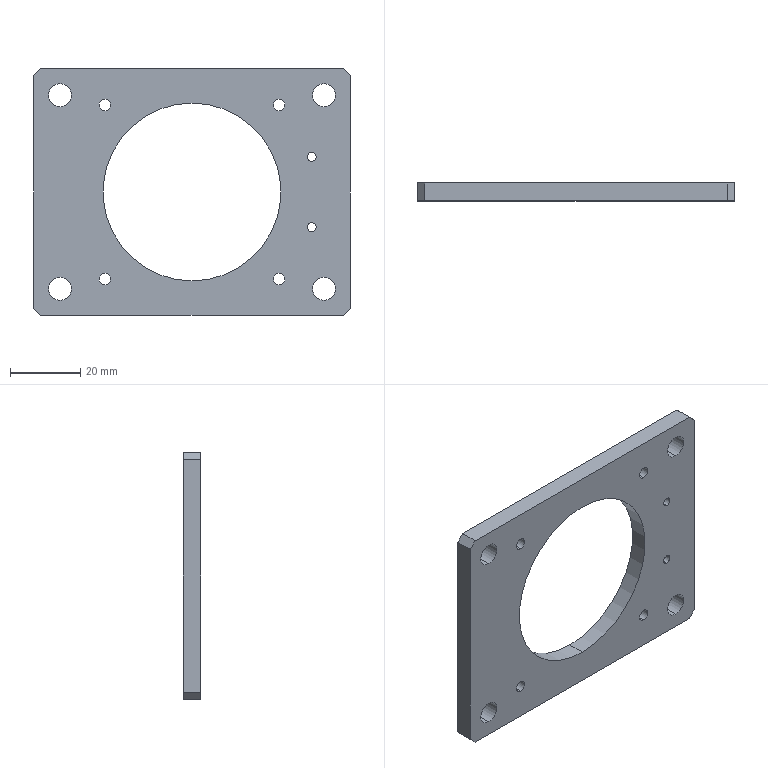Component | SolidWorks | H2020022-0411-1-1 | 1 solid | 32 faces | box 90 x 5 x 70 mm | volume 20561 mm3 | cylinder 22 | plane 10 | commonest cylinder face diameters 3.3 x8 6.5 x8 2.5 x4 50.5 x2 | material Stainless Steel304
STEP:
#1=COLOUR_RGB('',0.7922,0.8196,0.9333);
#2=FILL_AREA_STYLE_COLOUR('',#1);
#3=FILL_AREA_STYLE('',(#2));
#4=SURFACE_STYLE_FILL_AREA(#3);
#5=SURFACE_SIDE_STYLE('',(#4));
#6=SURFACE_STYLE_USAGE(.BOTH.,#5);
#7=PRESENTATION_STYLE_ASSIGNMENT((#6));
#8=CARTESIAN_POINT('',(0.1195,1.654,11.376));
#9=VERTEX_POINT('',#8);
#10=CARTESIAN_POINT('',(0.1195,1.654,11.474));
#11=VERTEX_POINT('',#10);
#12=CARTESIAN_POINT('',(0.1195,1.654,11.425));
#13=DIRECTION('',(0.,1.,-0.));
#14=DIRECTION('',(0.,0.,1.));
#15=AXIS2_PLACEMENT_3D('',#12,#13,#14);
#16=CIRCLE('',#15,0.04921);
#17=EDGE_CURVE('',#9,#11,#16,.T.);
#18=ORIENTED_EDGE('',*,*,#17,.F.);
#19=CARTESIAN_POINT('',(0.1195,1.851,11.376));
#20=VERTEX_POINT('',#19);
#21=CARTESIAN_POINT('',(0.1195,1.851,11.376));
#22=DIRECTION('',(0.,1.,-0.));
#23=VECTOR('',#22,39.37);
#24=LINE('',#21,#23);
#25=EDGE_CURVE('',#9,#20,#24,.T.);
#26=ORIENTED_EDGE('',*,*,#25,.T.);
#27=CARTESIAN_POINT('',(0.1195,1.851,11.474));
#28=VERTEX_POINT('',#27);
#29=CARTESIAN_POINT('',(0.1195,1.851,11.425));
#30=DIRECTION('',(0.,1.,-0.));
#31=DIRECTION('',(0.,0.,1.));
#32=AXIS2_PLACEMENT_3D('',#29,#30,#31);
#33=CIRCLE('',#32,0.04921);
#34=EDGE_CURVE('',#20,#28,#33,.T.);
#35=ORIENTED_EDGE('',*,*,#34,.T.);
#36=CARTESIAN_POINT('',(0.1195,1.851,11.474));
#37=DIRECTION('',(0.,1.,-0.));
#38=VECTOR('',#37,39.37);
#39=LINE('',#36,#38);
#40=EDGE_CURVE('',#11,#28,#39,.T.);
#41=ORIENTED_EDGE('',*,*,#40,.F.);
#42=EDGE_LOOP('',(#18,#26,#35,#41));
#43=FACE_OUTER_BOUND('',#42,.T.);
#44=CARTESIAN_POINT('',(0.1195,1.851,11.425));
#45=DIRECTION('',(0.,1.,-0.));
#46=DIRECTION('',(0.,0.,1.));
#47=AXIS2_PLACEMENT_3D('',#44,#45,#46);
#48=CYLINDRICAL_SURFACE('',#47,0.04921);
#49=ADVANCED_FACE('',(#43),#48,.F.);
#50=CARTESIAN_POINT('',(0.1195,1.654,10.588));
#51=VERTEX_POINT('',#50);
#52=CARTESIAN_POINT('',(0.1195,1.654,10.687));
#53=VERTEX_POINT('',#52);
#54=CARTESIAN_POINT('',(0.1195,1.654,10.638));
#55=DIRECTION('',(0.,1.,-0.));
#56=DIRECTION('',(0.,0.,1.));
#57=AXIS2_PLACEMENT_3D('',#54,#55,#56);
#58=CIRCLE('',#57,0.04921);
#59=EDGE_CURVE('',#51,#53,#58,.T.);
#60=ORIENTED_EDGE('',*,*,#59,.F.);
#61=CARTESIAN_POINT('',(0.1195,1.851,10.588));
#62=VERTEX_POINT('',#61);
#63=CARTESIAN_POINT('',(0.1195,1.851,10.588));
#64=DIRECTION('',(0.,1.,-0.));
#65=VECTOR('',#64,39.37);
#66=LINE('',#63,#65);
#67=EDGE_CURVE('',#51,#62,#66,.T.);
#68=ORIENTED_EDGE('',*,*,#67,.T.);
#69=CARTESIAN_POINT('',(0.1195,1.851,10.687));
#70=VERTEX_POINT('',#69);
#71=CARTESIAN_POINT('',(0.1195,1.851,10.638));
#72=DIRECTION('',(0.,1.,-0.));
#73=DIRECTION('',(0.,0.,1.));
#74=AXIS2_PLACEMENT_3D('',#71,#72,#73);
#75=CIRCLE('',#74,0.04921);
#76=EDGE_CURVE('',#62,#70,#75,.T.);
#77=ORIENTED_EDGE('',*,*,#76,.T.);
#78=CARTESIAN_POINT('',(0.1195,1.851,10.687));
#79=DIRECTION('',(0.,1.,-0.));
#80=VECTOR('',#79,39.37);
#81=LINE('',#78,#80);
#82=EDGE_CURVE('',#53,#70,#81,.T.);
#83=ORIENTED_EDGE('',*,*,#82,.F.);
#84=EDGE_LOOP('',(#60,#68,#77,#83));
#85=FACE_OUTER_BOUND('',#84,.T.);
#86=CARTESIAN_POINT('',(0.1195,1.851,10.638));
#87=DIRECTION('',(0.,1.,-0.));
#88=DIRECTION('',(0.,0.,1.));
#89=AXIS2_PLACEMENT_3D('',#86,#87,#88);
#90=CYLINDRICAL_SURFACE('',#89,0.04921);
#91=ADVANCED_FACE('',(#85),#90,.F.);
#92=CARTESIAN_POINT('',(-2.193,1.654,12.071));
#93=VERTEX_POINT('',#92);
#94=CARTESIAN_POINT('',(-2.193,1.654,11.941));
#95=VERTEX_POINT('',#94);
#96=CARTESIAN_POINT('',(-2.193,1.654,12.006));
#97=DIRECTION('',(-0.,-1.,0.));
#98=DIRECTION('',(0.,0.,-1.));
#99=AXIS2_PLACEMENT_3D('',#96,#97,#98);
#100=CIRCLE('',#99,0.06496);
#101=EDGE_CURVE('',#93,#95,#100,.T.);
#102=ORIENTED_EDGE('',*,*,#101,.T.);
#103=CARTESIAN_POINT('',(-2.193,1.851,11.941));
#104=VERTEX_POINT('',#103);
#105=CARTESIAN_POINT('',(-2.193,1.851,11.941));
#106=DIRECTION('',(0.,1.,-0.));
#107=VECTOR('',#106,39.37);
#108=LINE('',#105,#107);
#109=EDGE_CURVE('',#95,#104,#108,.T.);
#110=ORIENTED_EDGE('',*,*,#109,.T.);
#111=CARTESIAN_POINT('',(-2.193,1.851,12.071));
#112=VERTEX_POINT('',#111);
#113=CARTESIAN_POINT('',(-2.193,1.851,12.006));
#114=DIRECTION('',(0.,1.,-0.));
#115=DIRECTION('',(0.,0.,1.));
#116=AXIS2_PLACEMENT_3D('',#113,#114,#115);
#117=CIRCLE('',#116,0.06496);
#118=EDGE_CURVE('',#104,#112,#117,.T.);
#119=ORIENTED_EDGE('',*,*,#118,.T.);
#120=CARTESIAN_POINT('',(-2.193,1.851,12.071));
#121=DIRECTION('',(0.,1.,-0.));
#122=VECTOR('',#121,39.37);
#123=LINE('',#120,#122);
#124=EDGE_CURVE('',#93,#112,#123,.T.);
#125=ORIENTED_EDGE('',*,*,#124,.F.);
#126=EDGE_LOOP('',(#102,#110,#119,#125));
#127=FACE_OUTER_BOUND('',#126,.T.);
#128=CARTESIAN_POINT('',(-2.193,1.851,12.006));
#129=DIRECTION('',(0.,1.,-0.));
#130=DIRECTION('',(0.,0.,1.));
#131=AXIS2_PLACEMENT_3D('',#128,#129,#130);
#132=CYLINDRICAL_SURFACE('',#131,0.06496);
#133=ADVANCED_FACE('',(#127),#132,.F.);
#134=CARTESIAN_POINT('',(-2.193,1.654,10.122));
#135=VERTEX_POINT('',#134);
#136=CARTESIAN_POINT('',(-2.193,1.654,9.992));
#137=VERTEX_POINT('',#136);
#138=CARTESIAN_POINT('',(-2.193,1.654,10.057));
#139=DIRECTION('',(-0.,-1.,0.));
#140=DIRECTION('',(0.,0.,-1.));
#141=AXIS2_PLACEMENT_3D('',#138,#139,#140);
#142=CIRCLE('',#141,0.06496);
#143=EDGE_CURVE('',#135,#137,#142,.T.);
#144=ORIENTED_EDGE('',*,*,#143,.T.);
#145=CARTESIAN_POINT('',(-2.193,1.851,9.992));
#146=VERTEX_POINT('',#145);
#147=CARTESIAN_POINT('',(-2.193,1.851,9.992));
#148=DIRECTION('',(0.,1.,-0.));
#149=VECTOR('',#148,39.37);
#150=LINE('',#147,#149);
#151=EDGE_CURVE('',#137,#146,#150,.T.);
#152=ORIENTED_EDGE('',*,*,#151,.T.);
#153=CARTESIAN_POINT('',(-2.193,1.851,10.122));
#154=VERTEX_POINT('',#153);
#155=CARTESIAN_POINT('',(-2.193,1.851,10.057));
#156=DIRECTION('',(0.,1.,-0.));
#157=DIRECTION('',(0.,0.,1.));
#158=AXIS2_PLACEMENT_3D('',#155,#156,#157);
#159=CIRCLE('',#158,0.06496);
#160=EDGE_CURVE('',#146,#154,#159,.T.);
#161=ORIENTED_EDGE('',*,*,#160,.T.);
#162=CARTESIAN_POINT('',(-2.193,1.851,10.122));
#163=DIRECTION('',(0.,1.,-0.));
#164=VECTOR('',#163,39.37);
#165=LINE('',#162,#164);
#166=EDGE_CURVE('',#135,#154,#165,.T.);
#167=ORIENTED_EDGE('',*,*,#166,.F.);
#168=EDGE_LOOP('',(#144,#152,#161,#167));
#169=FACE_OUTER_BOUND('',#168,.T.);
#170=CARTESIAN_POINT('',(-2.193,1.851,10.057));
#171=DIRECTION('',(0.,1.,-0.));
#172=DIRECTION('',(0.,0.,1.));
#173=AXIS2_PLACEMENT_3D('',#170,#171,#172);
#174=CYLINDRICAL_SURFACE('',#173,0.06496);
#175=ADVANCED_FACE('',(#169),#174,.F.);
#176=CARTESIAN_POINT('',(-0.2447,1.654,10.122));
#177=VERTEX_POINT('',#176);
#178=CARTESIAN_POINT('',(-0.2447,1.654,9.992));
#179=VERTEX_POINT('',#178);
#180=CARTESIAN_POINT('',(-0.2447,1.654,10.057));
#181=DIRECTION('',(-0.,-1.,0.));
#182=DIRECTION('',(0.,0.,-1.));
#183=AXIS2_PLACEMENT_3D('',#180,#181,#182);
#184=CIRCLE('',#183,0.06496);
#185=EDGE_CURVE('',#177,#179,#184,.T.);
#186=ORIENTED_EDGE('',*,*,#185,.T.);
#187=CARTESIAN_POINT('',(-0.2447,1.851,9.992));
#188=VERTEX_POINT('',#187);
#189=CARTESIAN_POINT('',(-0.2447,1.851,9.992));
#190=DIRECTION('',(0.,1.,-0.));
#191=VECTOR('',#190,39.37);
#192=LINE('',#189,#191);
#193=EDGE_CURVE('',#179,#188,#192,.T.);
#194=ORIENTED_EDGE('',*,*,#193,.T.);
#195=CARTESIAN_POINT('',(-0.2447,1.851,10.122));
#196=VERTEX_POINT('',#195);
#197=CARTESIAN_POINT('',(-0.2447,1.851,10.057));
#198=DIRECTION('',(0.,1.,-0.));
#199=DIRECTION('',(0.,0.,1.));
#200=AXIS2_PLACEMENT_3D('',#197,#198,#199);
#201=CIRCLE('',#200,0.06496);
#202=EDGE_CURVE('',#188,#196,#201,.T.);
#203=ORIENTED_EDGE('',*,*,#202,.T.);
#204=CARTESIAN_POINT('',(-0.2447,1.851,10.122));
#205=DIRECTION('',(0.,1.,-0.));
#206=VECTOR('',#205,39.37);
#207=LINE('',#204,#206);
#208=EDGE_CURVE('',#177,#196,#207,.T.);
#209=ORIENTED_EDGE('',*,*,#208,.F.);
#210=EDGE_LOOP('',(#186,#194,#203,#209));
#211=FACE_OUTER_BOUND('',#210,.T.);
#212=CARTESIAN_POINT('',(-0.2447,1.851,10.057));
#213=DIRECTION('',(0.,1.,-0.));
#214=DIRECTION('',(0.,0.,1.));
#215=AXIS2_PLACEMENT_3D('',#212,#213,#214);
#216=CYLINDRICAL_SURFACE('',#215,0.06496);
#217=ADVANCED_FACE('',(#211),#216,.F.);
#218=CARTESIAN_POINT('',(-0.2447,1.654,12.071));
#219=VERTEX_POINT('',#218);
#220=CARTESIAN_POINT('',(-0.2447,1.654,11.941));
#221=VERTEX_POINT('',#220);
#222=CARTESIAN_POINT('',(-0.2447,1.654,12.006));
#223=DIRECTION('',(-0.,-1.,0.));
#224=DIRECTION('',(0.,0.,-1.));
#225=AXIS2_PLACEMENT_3D('',#222,#223,#224);
#226=CIRCLE('',#225,0.06496);
#227=EDGE_CURVE('',#219,#221,#226,.T.);
#228=ORIENTED_EDGE('',*,*,#227,.T.);
#229=CARTESIAN_POINT('',(-0.2447,1.851,11.941));
#230=VERTEX_POINT('',#229);
#231=CARTESIAN_POINT('',(-0.2447,1.851,11.941));
#232=DIRECTION('',(0.,1.,-0.));
#233=VECTOR('',#232,39.37);
#234=LINE('',#231,#233);
#235=EDGE_CURVE('',#221,#230,#234,.T.);
#236=ORIENTED_EDGE('',*,*,#235,.T.);
#237=CARTESIAN_POINT('',(-0.2447,1.851,12.071));
#238=VERTEX_POINT('',#237);
#239=CARTESIAN_POINT('',(-0.2447,1.851,12.006));
#240=DIRECTION('',(0.,1.,-0.));
#241=DIRECTION('',(0.,0.,1.));
#242=AXIS2_PLACEMENT_3D('',#239,#240,#241);
#243=CIRCLE('',#242,0.06496);
#244=EDGE_CURVE('',#230,#238,#243,.T.);
#245=ORIENTED_EDGE('',*,*,#244,.T.);
#246=CARTESIAN_POINT('',(-0.2447,1.851,12.071));
#247=DIRECTION('',(0.,1.,-0.));
#248=VECTOR('',#247,39.37);
#249=LINE('',#246,#248);
#250=EDGE_CURVE('',#219,#238,#249,.T.);
#251=ORIENTED_EDGE('',*,*,#250,.F.);
#252=EDGE_LOOP('',(#228,#236,#245,#251));
#253=FACE_OUTER_BOUND('',#252,.T.);
#254=CARTESIAN_POINT('',(-0.2447,1.851,12.006));
#255=DIRECTION('',(0.,1.,-0.));
#256=DIRECTION('',(0.,0.,1.));
#257=AXIS2_PLACEMENT_3D('',#254,#255,#256);
#258=CYLINDRICAL_SURFACE('',#257,0.06496);
#259=ADVANCED_FACE('',(#253),#258,.F.);
#260=CARTESIAN_POINT('',(-2.695,1.851,12.242));
#261=VERTEX_POINT('',#260);
#262=CARTESIAN_POINT('',(-2.695,1.851,11.986));
#263=VERTEX_POINT('',#262);
#264=CARTESIAN_POINT('',(-2.695,1.851,12.114));
#265=DIRECTION('',(-0.,-1.,0.));
#266=DIRECTION('',(0.,0.,-1.));
#267=AXIS2_PLACEMENT_3D('',#264,#265,#266);
#268=CIRCLE('',#267,0.128);
#269=EDGE_CURVE('',#261,#263,#268,.T.);
#270=ORIENTED_EDGE('',*,*,#269,.F.);
#271=CARTESIAN_POINT('',(-2.695,1.654,12.242));
#272=VERTEX_POINT('',#271);
#273=CARTESIAN_POINT('',(-2.695,1.654,12.242));
#274=DIRECTION('',(-0.,-1.,0.));
#275=VECTOR('',#274,39.37);
#276=LINE('',#273,#275);
#277=EDGE_CURVE('',#261,#272,#276,.T.);
#278=ORIENTED_EDGE('',*,*,#277,.T.);
#279=CARTESIAN_POINT('',(-2.695,1.654,11.986));
#280=VERTEX_POINT('',#279);
#281=CARTESIAN_POINT('',(-2.695,1.654,12.114));
#282=DIRECTION('',(-0.,-1.,0.));
#283=DIRECTION('',(0.,0.,-1.));
#284=AXIS2_PLACEMENT_3D('',#281,#282,#283);
#285=CIRCLE('',#284,0.128);
#286=EDGE_CURVE('',#272,#280,#285,.T.);
#287=ORIENTED_EDGE('',*,*,#286,.T.);
#288=CARTESIAN_POINT('',(-2.695,1.654,11.986));
#289=DIRECTION('',(-0.,-1.,0.));
#290=VECTOR('',#289,39.37);
#291=LINE('',#288,#290);
#292=EDGE_CURVE('',#263,#280,#291,.T.);
#293=ORIENTED_EDGE('',*,*,#292,.F.);
#294=EDGE_LOOP('',(#270,#278,#287,#293));
#295=FACE_OUTER_BOUND('',#294,.T.);
#296=CARTESIAN_POINT('',(-2.695,1.654,12.114));
#297=DIRECTION('',(-0.,-1.,0.));
#298=DIRECTION('',(0.,0.,-1.));
#299=AXIS2_PLACEMENT_3D('',#296,#297,#298);
#300=CYLINDRICAL_SURFACE('',#299,0.128);
#301=ADVANCED_FACE('',(#295),#300,.F.);
#302=CARTESIAN_POINT('',(-2.695,1.851,10.077));
#303=VERTEX_POINT('',#302);
#304=CARTESIAN_POINT('',(-2.695,1.851,9.821));
#305=VERTEX_POINT('',#304);
#306=CARTESIAN_POINT('',(-2.695,1.851,9.949));
#307=DIRECTION('',(-0.,-1.,0.));
#308=DIRECTION('',(0.,0.,-1.));
#309=AXIS2_PLACEMENT_3D('',#306,#307,#308);
#310=CIRCLE('',#309,0.128);
#311=EDGE_CURVE('',#303,#305,#310,.T.);
#312=ORIENTED_EDGE('',*,*,#311,.F.);
#313=CARTESIAN_POINT('',(-2.695,1.654,10.077));
#314=VERTEX_POINT('',#313);
#315=CARTESIAN_POINT('',(-2.695,1.654,10.077));
#316=DIRECTION('',(-0.,-1.,0.));
#317=VECTOR('',#316,39.37);
#318=LINE('',#315,#317);
#319=EDGE_CURVE('',#303,#314,#318,.T.);
#320=ORIENTED_EDGE('',*,*,#319,.T.);
#321=CARTESIAN_POINT('',(-2.695,1.654,9.821));
#322=VERTEX_POINT('',#321);
#323=CARTESIAN_POINT('',(-2.695,1.654,9.949));
#324=DIRECTION('',(-0.,-1.,0.));
#325=DIRECTION('',(0.,0.,-1.));
#326=AXIS2_PLACEMENT_3D('',#323,#324,#325);
#327=CIRCLE('',#326,0.128);
#328=EDGE_CURVE('',#314,#322,#327,.T.);
#329=ORIENTED_EDGE('',*,*,#328,.T.);
#330=CARTESIAN_POINT('',(-2.695,1.654,9.821));
#331=DIRECTION('',(-0.,-1.,0.));
#332=VECTOR('',#331,39.37);
#333=LINE('',#330,#332);
#334=EDGE_CURVE('',#305,#322,#333,.T.);
#335=ORIENTED_EDGE('',*,*,#334,.F.);
#336=EDGE_LOOP('',(#312,#320,#329,#335));
#337=FACE_OUTER_BOUND('',#336,.T.);
#338=CARTESIAN_POINT('',(-2.695,1.654,9.949));
#339=DIRECTION('',(-0.,-1.,0.));
#340=DIRECTION('',(0.,0.,-1.));
#341=AXIS2_PLACEMENT_3D('',#338,#339,#340);
#342=CYLINDRICAL_SURFACE('',#341,0.128);
#343=ADVANCED_FACE('',(#337),#342,.F.);
#344=CARTESIAN_POINT('',(0.2573,1.851,10.077));
#345=VERTEX_POINT('',#344);
#346=CARTESIAN_POINT('',(0.2573,1.851,9.821));
#347=VERTEX_POINT('',#346);
#348=CARTESIAN_POINT('',(0.2573,1.851,9.949));
#349=DIRECTION('',(-0.,-1.,0.));
#350=DIRECTION('',(0.,0.,-1.));
#351=AXIS2_PLACEMENT_3D('',#348,#349,#350);
#352=CIRCLE('',#351,0.128);
#353=EDGE_CURVE('',#345,#347,#352,.T.);
#354=ORIENTED_EDGE('',*,*,#353,.F.);
#355=CARTESIAN_POINT('',(0.2573,1.654,10.077));
#356=VERTEX_POINT('',#355);
#357=CARTESIAN_POINT('',(0.2573,1.654,10.077));
#358=DIRECTION('',(-0.,-1.,0.));
#359=VECTOR('',#358,39.37);
#360=LINE('',#357,#359);
#361=EDGE_CURVE('',#345,#356,#360,.T.);
#362=ORIENTED_EDGE('',*,*,#361,.T.);
#363=CARTESIAN_POINT('',(0.2573,1.654,9.821));
#364=VERTEX_POINT('',#363);
#365=CARTESIAN_POINT('',(0.2573,1.654,9.949));
#366=DIRECTION('',(-0.,-1.,0.));
#367=DIRECTION('',(0.,0.,-1.));
#368=AXIS2_PLACEMENT_3D('',#365,#366,#367);
#369=CIRCLE('',#368,0.128);
#370=EDGE_CURVE('',#356,#364,#369,.T.);
#371=ORIENTED_EDGE('',*,*,#370,.T.);
#372=CARTESIAN_POINT('',(0.2573,1.654,9.821));
#373=DIRECTION('',(-0.,-1.,0.));
#374=VECTOR('',#373,39.37);
#375=LINE('',#372,#374);
#376=EDGE_CURVE('',#347,#364,#375,.T.);
#377=ORIENTED_EDGE('',*,*,#376,.F.);
#378=EDGE_LOOP('',(#354,#362,#371,#377));
#379=FACE_OUTER_BOUND('',#378,.T.);
#380=CARTESIAN_POINT('',(0.2573,1.654,9.949));
#381=DIRECTION('',(-0.,-1.,0.));
#382=DIRECTION('',(0.,0.,-1.));
#383=AXIS2_PLACEMENT_3D('',#380,#381,#382);
#384=CYLINDRICAL_SURFACE('',#383,0.128);
#385=ADVANCED_FACE('',(#379),#384,.F.);
#386=CARTESIAN_POINT('',(0.2573,1.851,12.242));
#387=VERTEX_POINT('',#386);
#388=CARTESIAN_POINT('',(0.2573,1.851,11.986));
#389=VERTEX_POINT('',#388);
#390=CARTESIAN_POINT('',(0.2573,1.851,12.114));
#391=DIRECTION('',(-0.,-1.,0.));
#392=DIRECTION('',(0.,0.,-1.));
#393=AXIS2_PLACEMENT_3D('',#390,#391,#392);
#394=CIRCLE('',#393,0.128);
#395=EDGE_CURVE('',#387,#389,#394,.T.);
#396=ORIENTED_EDGE('',*,*,#395,.F.);
#397=CARTESIAN_POINT('',(0.2573,1.654,12.242));
#398=VERTEX_POINT('',#397);
#399=CARTESIAN_POINT('',(0.2573,1.654,12.242));
#400=DIRECTION('',(-0.,-1.,0.));
#401=VECTOR('',#400,39.37);
#402=LINE('',#399,#401);
#403=EDGE_CURVE('',#387,#398,#402,.T.);
#404=ORIENTED_EDGE('',*,*,#403,.T.);
#405=CARTESIAN_POINT('',(0.2573,1.654,11.986));
#406=VERTEX_POINT('',#405);
#407=CARTESIAN_POINT('',(0.2573,1.654,12.114));
#408=DIRECTION('',(-0.,-1.,0.));
#409=DIRECTION('',(0.,0.,-1.));
#410=AXIS2_PLACEMENT_3D('',#407,#408,#409);
#411=CIRCLE('',#410,0.128);
#412=EDGE_CURVE('',#398,#406,#411,.T.);
#413=ORIENTED_EDGE('',*,*,#412,.T.);
#414=CARTESIAN_POINT('',(0.2573,1.654,11.986));
#415=DIRECTION('',(-0.,-1.,0.));
#416=VECTOR('',#415,39.37);
#417=LINE('',#414,#416);
#418=EDGE_CURVE('',#389,#406,#417,.T.);
#419=ORIENTED_EDGE('',*,*,#418,.F.);
#420=EDGE_LOOP('',(#396,#404,#413,#419));
#421=FACE_OUTER_BOUND('',#420,.T.);
#422=CARTESIAN_POINT('',(0.2573,1.654,12.114));
#423=DIRECTION('',(-0.,-1.,0.));
#424=DIRECTION('',(0.,0.,-1.));
#425=AXIS2_PLACEMENT_3D('',#422,#423,#424);
#426=CYLINDRICAL_SURFACE('',#425,0.128);
#427=ADVANCED_FACE('',(#421),#426,.F.);
#428=CARTESIAN_POINT('',(-1.219,1.654,10.037));
#429=VERTEX_POINT('',#428);
#430=CARTESIAN_POINT('',(-1.219,1.654,12.025));
#431=VERTEX_POINT('',#430);
#432=CARTESIAN_POINT('',(-1.219,1.654,11.031));
#433=DIRECTION('',(0.,1.,-0.));
#434=DIRECTION('',(0.,0.,1.));
#435=AXIS2_PLACEMENT_3D('',#432,#433,#434);
#436=CIRCLE('',#435,0.9941);
#437=EDGE_CURVE('',#429,#431,#436,.T.);
#438=ORIENTED_EDGE('',*,*,#437,.F.);
#439=CARTESIAN_POINT('',(-1.219,1.851,10.037));
#440=VERTEX_POINT('',#439);
#441=CARTESIAN_POINT('',(-1.219,1.654,10.037));
#442=DIRECTION('',(0.,1.,-0.));
#443=VECTOR('',#442,39.37);
#444=LINE('',#441,#443);
#445=EDGE_CURVE('',#429,#440,#444,.T.);
#446=ORIENTED_EDGE('',*,*,#445,.T.);
#447=CARTESIAN_POINT('',(-1.219,1.851,12.025));
#448=VERTEX_POINT('',#447);
#449=CARTESIAN_POINT('',(-1.219,1.851,11.031));
#450=DIRECTION('',(0.,1.,-0.));
#451=DIRECTION('',(0.,0.,1.));
#452=AXIS2_PLACEMENT_3D('',#449,#450,#451);
#453=CIRCLE('',#452,0.9941);
#454=EDGE_CURVE('',#440,#448,#453,.T.);
#455=ORIENTED_EDGE('',*,*,#454,.T.);
#456=CARTESIAN_POINT('',(-1.219,1.654,12.025));
#457=DIRECTION('',(0.,1.,-0.));
#458=VECTOR('',#457,39.37);
#459=LINE('',#456,#458);
#460=EDGE_CURVE('',#431,#448,#459,.T.);
#461=ORIENTED_EDGE('',*,*,#460,.F.);
#462=EDGE_LOOP('',(#438,#446,#455,#461));
#463=FACE_OUTER_BOUND('',#462,.T.);
#464=CARTESIAN_POINT('',(-1.219,1.654,11.031));
#465=DIRECTION('',(0.,1.,-0.));
#466=DIRECTION('',(0.,0.,1.));
#467=AXIS2_PLACEMENT_3D('',#464,#465,#466);
#468=CYLINDRICAL_SURFACE('',#467,0.9941);
#469=ADVANCED_FACE('',(#463),#468,.F.);
#470=CARTESIAN_POINT('',(0.1195,1.851,11.425));
#471=DIRECTION('',(0.,1.,-0.));
#472=DIRECTION('',(0.,0.,1.));
#473=AXIS2_PLACEMENT_3D('',#470,#471,#472);
#474=CIRCLE('',#473,0.04921);
#475=EDGE_CURVE('',#28,#20,#474,.T.);
#476=ORIENTED_EDGE('',*,*,#475,.F.);
#477=ORIENTED_EDGE('',*,*,#34,.F.);
#478=EDGE_LOOP('',(#476,#477));
#479=FACE_BOUND('',#478,.T.);
#480=CARTESIAN_POINT('',(0.1195,1.851,10.638));
#481=DIRECTION('',(0.,1.,-0.));
#482=DIRECTION('',(0.,0.,1.));
#483=AXIS2_PLACEMENT_3D('',#480,#481,#482);
#484=CIRCLE('',#483,0.04921);
#485=EDGE_CURVE('',#70,#62,#484,.T.);
#486=ORIENTED_EDGE('',*,*,#485,.F.);
#487=ORIENTED_EDGE('',*,*,#76,.F.);
#488=EDGE_LOOP('',(#486,#487));
#489=FACE_BOUND('',#488,.T.);
#490=CARTESIAN_POINT('',(-2.193,1.851,10.057));
#491=DIRECTION('',(0.,1.,-0.));
#492=DIRECTION('',(0.,0.,1.));
#493=AXIS2_PLACEMENT_3D('',#490,#491,#492);
#494=CIRCLE('',#493,0.06496);
#495=EDGE_CURVE('',#154,#146,#494,.T.);
#496=ORIENTED_EDGE('',*,*,#495,.F.);
#497=ORIENTED_EDGE('',*,*,#160,.F.);
#498=EDGE_LOOP('',(#496,#497));
#499=FACE_BOUND('',#498,.T.);
#500=CARTESIAN_POINT('',(-0.2447,1.851,10.057));
#501=DIRECTION('',(0.,1.,-0.));
#502=DIRECTION('',(0.,0.,1.));
#503=AXIS2_PLACEMENT_3D('',#500,#501,#502);
#504=CIRCLE('',#503,0.06496);
#505=EDGE_CURVE('',#196,#188,#504,.T.);
#506=ORIENTED_EDGE('',*,*,#505,.F.);
#507=ORIENTED_EDGE('',*,*,#202,.F.);
#508=EDGE_LOOP('',(#506,#507));
#509=FACE_BOUND('',#508,.T.);
#510=CARTESIAN_POINT('',(-0.2447,1.851,12.006));
#511=DIRECTION('',(0.,1.,-0.));
#512=DIRECTION('',(0.,0.,1.));
#513=AXIS2_PLACEMENT_3D('',#510,#511,#512);
#514=CIRCLE('',#513,0.06496);
#515=EDGE_CURVE('',#238,#230,#514,.T.);
#516=ORIENTED_EDGE('',*,*,#515,.F.);
#517=ORIENTED_EDGE('',*,*,#244,.F.);
#518=EDGE_LOOP('',(#516,#517));
#519=FACE_BOUND('',#518,.T.);
#520=CARTESIAN_POINT('',(-2.695,1.851,12.114));
#521=DIRECTION('',(-0.,-1.,0.));
#522=DIRECTION('',(0.,0.,-1.));
#523=AXIS2_PLACEMENT_3D('',#520,#521,#522);
#524=CIRCLE('',#523,0.128);
#525=EDGE_CURVE('',#263,#261,#524,.T.);
#526=ORIENTED_EDGE('',*,*,#525,.T.);
#527=ORIENTED_EDGE('',*,*,#269,.T.);
#528=EDGE_LOOP('',(#526,#527));
#529=FACE_BOUND('',#528,.T.);
#530=CARTESIAN_POINT('',(-2.695,1.851,9.949));
#531=DIRECTION('',(-0.,-1.,0.));
#532=DIRECTION('',(0.,0.,-1.));
#533=AXIS2_PLACEMENT_3D('',#530,#531,#532);
#534=CIRCLE('',#533,0.128);
#535=EDGE_CURVE('',#305,#303,#534,.T.);
#536=ORIENTED_EDGE('',*,*,#535,.T.);
#537=ORIENTED_EDGE('',*,*,#311,.T.);
#538=EDGE_LOOP('',(#536,#537));
#539=FACE_BOUND('',#538,.T.);
#540=CARTESIAN_POINT('',(0.2573,1.851,9.949));
#541=DIRECTION('',(-0.,-1.,0.));
#542=DIRECTION('',(0.,0.,-1.));
#543=AXIS2_PLACEMENT_3D('',#540,#541,#542);
#544=CIRCLE('',#543,0.128);
#545=EDGE_CURVE('',#347,#345,#544,.T.);
#546=ORIENTED_EDGE('',*,*,#545,.T.);
#547=ORIENTED_EDGE('',*,*,#353,.T.);
#548=EDGE_LOOP('',(#546,#547));
#549=FACE_BOUND('',#548,.T.);
#550=CARTESIAN_POINT('',(0.2573,1.851,12.114));
#551=DIRECTION('',(-0.,-1.,0.));
#552=DIRECTION('',(0.,0.,-1.));
#553=AXIS2_PLACEMENT_3D('',#550,#551,#552);
#554=CIRCLE('',#553,0.128);
#555=EDGE_CURVE('',#389,#387,#554,.T.);
#556=ORIENTED_EDGE('',*,*,#555,.T.);
#557=ORIENTED_EDGE('',*,*,#395,.T.);
#558=EDGE_LOOP('',(#556,#557));
#559=FACE_BOUND('',#558,.T.);
#560=CARTESIAN_POINT('',(-1.219,1.851,11.031));
#561=DIRECTION('',(0.,1.,-0.));
#562=DIRECTION('',(0.,0.,1.));
#563=AXIS2_PLACEMENT_3D('',#560,#561,#562);
#564=CIRCLE('',#563,0.9941);
#565=EDGE_CURVE('',#448,#440,#564,.T.);
#566=ORIENTED_EDGE('',*,*,#565,.F.);
#567=ORIENTED_EDGE('',*,*,#454,.F.);
#568=EDGE_LOOP('',(#566,#567));
#569=FACE_BOUND('',#568,.T.);
#570=CARTESIAN_POINT('',(-2.991,1.851,9.732));
#571=VERTEX_POINT('',#570);
#572=CARTESIAN_POINT('',(-2.991,1.851,12.331));
#573=VERTEX_POINT('',#572);
#574=CARTESIAN_POINT('',(-2.991,1.851,9.653));
#575=DIRECTION('',(0.,0.,1.));
#576=VECTOR('',#575,39.37);
#577=LINE('',#574,#576);
#578=EDGE_CURVE('',#571,#573,#577,.T.);
#579=ORIENTED_EDGE('',*,*,#578,.T.);
#580=CARTESIAN_POINT('',(-2.912,1.851,12.409));
#581=VERTEX_POINT('',#580);
#582=CARTESIAN_POINT('',(-2.912,1.851,12.409));
#583=DIRECTION('',(0.7071,-0.,0.7071));
#584=VECTOR('',#583,39.37);
#585=LINE('',#582,#584);
#586=EDGE_CURVE('',#573,#581,#585,.T.);
#587=ORIENTED_EDGE('',*,*,#586,.T.);
#588=CARTESIAN_POINT('',(0.4738,1.851,12.409));
#589=VERTEX_POINT('',#588);
#590=CARTESIAN_POINT('',(-2.991,1.851,12.409));
#591=DIRECTION('',(1.,-0.,0.));
#592=VECTOR('',#591,39.37);
#593=LINE('',#590,#592);
#594=EDGE_CURVE('',#581,#589,#593,.T.);
#595=ORIENTED_EDGE('',*,*,#594,.T.);
#596=CARTESIAN_POINT('',(0.5526,1.851,12.331));
#597=VERTEX_POINT('',#596);
#598=CARTESIAN_POINT('',(0.5526,1.851,12.331));
#599=DIRECTION('',(0.7071,-0.,-0.7071));
#600=VECTOR('',#599,39.37);
#601=LINE('',#598,#600);
#602=EDGE_CURVE('',#589,#597,#601,.T.);
#603=ORIENTED_EDGE('',*,*,#602,.T.);
#604=CARTESIAN_POINT('',(0.5526,1.851,9.732));
#605=VERTEX_POINT('',#604);
#606=CARTESIAN_POINT('',(0.5526,1.851,9.653));
#607=DIRECTION('',(-0.,-0.,-1.));
#608=VECTOR('',#607,39.37);
#609=LINE('',#606,#608);
#610=EDGE_CURVE('',#597,#605,#609,.T.);
#611=ORIENTED_EDGE('',*,*,#610,.T.);
#612=CARTESIAN_POINT('',(0.4738,1.851,9.653));
#613=VERTEX_POINT('',#612);
#614=CARTESIAN_POINT('',(0.4738,1.851,9.653));
#615=DIRECTION('',(-0.7071,0.,-0.7071));
#616=VECTOR('',#615,39.37);
#617=LINE('',#614,#616);
#618=EDGE_CURVE('',#605,#613,#617,.T.);
#619=ORIENTED_EDGE('',*,*,#618,.T.);
#620=CARTESIAN_POINT('',(-2.912,1.851,9.653));
#621=VERTEX_POINT('',#620);
#622=CARTESIAN_POINT('',(-2.991,1.851,9.653));
#623=DIRECTION('',(-1.,0.,-0.));
#624=VECTOR('',#623,39.37);
#625=LINE('',#622,#624);
#626=EDGE_CURVE('',#613,#621,#625,.T.);
#627=ORIENTED_EDGE('',*,*,#626,.T.);
#628=CARTESIAN_POINT('',(-2.991,1.851,9.732));
#629=DIRECTION('',(-0.7071,0.,0.7071));
#630=VECTOR('',#629,39.37);
#631=LINE('',#628,#630);
#632=EDGE_CURVE('',#621,#571,#631,.T.);
#633=ORIENTED_EDGE('',*,*,#632,.T.);
#634=EDGE_LOOP('',(#579,#587,#595,#603,#611,#619,#627,#633));
#635=FACE_OUTER_BOUND('',#634,.T.);
#636=CARTESIAN_POINT('',(-2.193,1.851,12.006));
#637=DIRECTION('',(0.,1.,-0.));
#638=DIRECTION('',(0.,0.,1.));
#639=AXIS2_PLACEMENT_3D('',#636,#637,#638);
#640=CIRCLE('',#639,0.06496);
#641=EDGE_CURVE('',#112,#104,#640,.T.);
#642=ORIENTED_EDGE('',*,*,#641,.F.);
#643=ORIENTED_EDGE('',*,*,#118,.F.);
#644=EDGE_LOOP('',(#642,#643));
#645=FACE_BOUND('',#644,.T.);
#646=CARTESIAN_POINT('',(-2.991,1.851,9.653));
#647=DIRECTION('',(-0.,-1.,0.));
#648=DIRECTION('',(-0.,-0.,-1.));
#649=AXIS2_PLACEMENT_3D('',#646,#647,#648);
#650=PLANE('',#649);
#651=ADVANCED_FACE('',(#479,#489,#499,#509,#519,#529,#539,#549,#559,#569,#635,#645),#650,.F.);
#652=CARTESIAN_POINT('',(0.4738,1.654,9.653));
#653=VERTEX_POINT('',#652);
#654=CARTESIAN_POINT('',(-2.912,1.654,9.653));
#655=VERTEX_POINT('',#654);
#656=CARTESIAN_POINT('',(-2.991,1.654,9.653));
#657=DIRECTION('',(-1.,0.,-0.));
#658=VECTOR('',#657,39.37);
#659=LINE('',#656,#658);
#660=EDGE_CURVE('',#653,#655,#659,.T.);
#661=ORIENTED_EDGE('',*,*,#660,.T.);
#662=CARTESIAN_POINT('',(-2.912,1.851,9.653));
#663=DIRECTION('',(0.,1.,-0.));
#664=VECTOR('',#663,39.37);
#665=LINE('',#662,#664);
#666=EDGE_CURVE('',#655,#621,#665,.T.);
#667=ORIENTED_EDGE('',*,*,#666,.T.);
#668=ORIENTED_EDGE('',*,*,#626,.F.);
#669=CARTESIAN_POINT('',(0.4738,1.851,9.653));
#670=DIRECTION('',(-0.,-1.,0.));
#671=VECTOR('',#670,39.37);
#672=LINE('',#669,#671);
#673=EDGE_CURVE('',#613,#653,#672,.T.);
#674=ORIENTED_EDGE('',*,*,#673,.T.);
#675=EDGE_LOOP('',(#661,#667,#668,#674));
#676=FACE_OUTER_BOUND('',#675,.T.);
#677=CARTESIAN_POINT('',(-2.991,1.851,9.653));
#678=DIRECTION('',(0.,0.,1.));
#679=DIRECTION('',(-0.,-1.,0.));
#680=AXIS2_PLACEMENT_3D('',#677,#678,#679);
#681=PLANE('',#680);
#682=ADVANCED_FACE('',(#676),#681,.F.);
#683=CARTESIAN_POINT('',(-2.991,1.654,9.732));
#684=VERTEX_POINT('',#683);
#685=CARTESIAN_POINT('',(-2.991,1.654,12.331));
#686=VERTEX_POINT('',#685);
#687=CARTESIAN_POINT('',(-2.991,1.654,9.653));
#688=DIRECTION('',(0.,0.,1.));
#689=VECTOR('',#688,39.37);
#690=LINE('',#687,#689);
#691=EDGE_CURVE('',#684,#686,#690,.T.);
#692=ORIENTED_EDGE('',*,*,#691,.T.);
#693=CARTESIAN_POINT('',(-2.991,1.851,12.331));
#694=DIRECTION('',(0.,1.,-0.));
#695=VECTOR('',#694,39.37);
#696=LINE('',#693,#695);
#697=EDGE_CURVE('',#686,#573,#696,.T.);
#698=ORIENTED_EDGE('',*,*,#697,.T.);
#699=ORIENTED_EDGE('',*,*,#578,.F.);
#700=CARTESIAN_POINT('',(-2.991,1.851,9.732));
#701=DIRECTION('',(-0.,-1.,0.));
#702=VECTOR('',#701,39.37);
#703=LINE('',#700,#702);
#704=EDGE_CURVE('',#571,#684,#703,.T.);
#705=ORIENTED_EDGE('',*,*,#704,.T.);
#706=EDGE_LOOP('',(#692,#698,#699,#705));
#707=FACE_OUTER_BOUND('',#706,.T.);
#708=CARTESIAN_POINT('',(-2.991,1.851,9.653));
#709=DIRECTION('',(1.,-0.,0.));
#710=DIRECTION('',(-0.,-0.,-1.));
#711=AXIS2_PLACEMENT_3D('',#708,#709,#710);
#712=PLANE('',#711);
#713=ADVANCED_FACE('',(#707),#712,.F.);
#714=ORIENTED_EDGE('',*,*,#594,.F.);
#715=CARTESIAN_POINT('',(-2.912,1.654,12.409));
#716=VERTEX_POINT('',#715);
#717=CARTESIAN_POINT('',(-2.912,1.851,12.409));
#718=DIRECTION('',(-0.,-1.,0.));
#719=VECTOR('',#718,39.37);
#720=LINE('',#717,#719);
#721=EDGE_CURVE('',#581,#716,#720,.T.);
#722=ORIENTED_EDGE('',*,*,#721,.T.);
#723=CARTESIAN_POINT('',(0.4738,1.654,12.409));
#724=VERTEX_POINT('',#723);
#725=CARTESIAN_POINT('',(-2.991,1.654,12.409));
#726=DIRECTION('',(1.,-0.,0.));
#727=VECTOR('',#726,39.37);
#728=LINE('',#725,#727);
#729=EDGE_CURVE('',#716,#724,#728,.T.);
#730=ORIENTED_EDGE('',*,*,#729,.T.);
#731=CARTESIAN_POINT('',(0.4738,1.851,12.409));
#732=DIRECTION('',(0.,1.,-0.));
#733=VECTOR('',#732,39.37);
#734=LINE('',#731,#733);
#735=EDGE_CURVE('',#724,#589,#734,.T.);
#736=ORIENTED_EDGE('',*,*,#735,.T.);
#737=EDGE_LOOP('',(#714,#722,#730,#736));
#738=FACE_OUTER_BOUND('',#737,.T.);
#739=CARTESIAN_POINT('',(-2.991,1.851,12.409));
#740=DIRECTION('',(-0.,-0.,-1.));
#741=DIRECTION('',(0.,1.,-0.));
#742=AXIS2_PLACEMENT_3D('',#739,#740,#741);
#743=PLANE('',#742);
#744=ADVANCED_FACE('',(#738),#743,.F.);
#745=ORIENTED_EDGE('',*,*,#610,.F.);
#746=CARTESIAN_POINT('',(0.5526,1.654,12.331));
#747=VERTEX_POINT('',#746);
#748=CARTESIAN_POINT('',(0.5526,1.851,12.331));
#749=DIRECTION('',(-0.,-1.,0.));
#750=VECTOR('',#749,39.37);
#751=LINE('',#748,#750);
#752=EDGE_CURVE('',#597,#747,#751,.T.);
#753=ORIENTED_EDGE('',*,*,#752,.T.);
#754=CARTESIAN_POINT('',(0.5526,1.654,9.732));
#755=VERTEX_POINT('',#754);
#756=CARTESIAN_POINT('',(0.5526,1.654,9.653));
#757=DIRECTION('',(-0.,-0.,-1.));
#758=VECTOR('',#757,39.37);
#759=LINE('',#756,#758);
#760=EDGE_CURVE('',#747,#755,#759,.T.);
#761=ORIENTED_EDGE('',*,*,#760,.T.);
#762=CARTESIAN_POINT('',(0.5526,1.851,9.732));
#763=DIRECTION('',(0.,1.,-0.));
#764=VECTOR('',#763,39.37);
#765=LINE('',#762,#764);
#766=EDGE_CURVE('',#755,#605,#765,.T.);
#767=ORIENTED_EDGE('',*,*,#766,.T.);
#768=EDGE_LOOP('',(#745,#753,#761,#767));
#769=FACE_OUTER_BOUND('',#768,.T.);
#770=CARTESIAN_POINT('',(0.5526,1.851,9.653));
#771=DIRECTION('',(-1.,0.,-0.));
#772=DIRECTION('',(0.,0.,1.));
#773=AXIS2_PLACEMENT_3D('',#770,#771,#772);
#774=PLANE('',#773);
#775=ADVANCED_FACE('',(#769),#774,.F.);
#776=CARTESIAN_POINT('',(0.1195,1.654,11.425));
#777=DIRECTION('',(0.,1.,-0.));
#778=DIRECTION('',(0.,0.,1.));
#779=AXIS2_PLACEMENT_3D('',#776,#777,#778);
#780=CIRCLE('',#779,0.04921);
#781=EDGE_CURVE('',#11,#9,#780,.T.);
#782=ORIENTED_EDGE('',*,*,#781,.T.);
#783=ORIENTED_EDGE('',*,*,#17,.T.);
#784=EDGE_LOOP('',(#782,#783));
#785=FACE_BOUND('',#784,.T.);
#786=CARTESIAN_POINT('',(0.1195,1.654,10.638));
#787=DIRECTION('',(0.,1.,-0.));
#788=DIRECTION('',(0.,0.,1.));
#789=AXIS2_PLACEMENT_3D('',#786,#787,#788);
#790=CIRCLE('',#789,0.04921);
#791=EDGE_CURVE('',#53,#51,#790,.T.);
#792=ORIENTED_EDGE('',*,*,#791,.T.);
#793=ORIENTED_EDGE('',*,*,#59,.T.);
#794=EDGE_LOOP('',(#792,#793));
#795=FACE_BOUND('',#794,.T.);
#796=ORIENTED_EDGE('',*,*,#101,.F.);
#797=CARTESIAN_POINT('',(-2.193,1.654,12.006));
#798=DIRECTION('',(-0.,-1.,0.));
#799=DIRECTION('',(0.,0.,-1.));
#800=AXIS2_PLACEMENT_3D('',#797,#798,#799);
#801=CIRCLE('',#800,0.06496);
#802=EDGE_CURVE('',#95,#93,#801,.T.);
#803=ORIENTED_EDGE('',*,*,#802,.F.);
#804=EDGE_LOOP('',(#796,#803));
#805=FACE_BOUND('',#804,.T.);
#806=ORIENTED_EDGE('',*,*,#143,.F.);
#807=CARTESIAN_POINT('',(-2.193,1.654,10.057));
#808=DIRECTION('',(-0.,-1.,0.));
#809=DIRECTION('',(0.,0.,-1.));
#810=AXIS2_PLACEMENT_3D('',#807,#808,#809);
#811=CIRCLE('',#810,0.06496);
#812=EDGE_CURVE('',#137,#135,#811,.T.);
#813=ORIENTED_EDGE('',*,*,#812,.F.);
#814=EDGE_LOOP('',(#806,#813));
#815=FACE_BOUND('',#814,.T.);
#816=ORIENTED_EDGE('',*,*,#185,.F.);
#817=CARTESIAN_POINT('',(-0.2447,1.654,10.057));
#818=DIRECTION('',(-0.,-1.,0.));
#819=DIRECTION('',(0.,0.,-1.));
#820=AXIS2_PLACEMENT_3D('',#817,#818,#819);
#821=CIRCLE('',#820,0.06496);
#822=EDGE_CURVE('',#179,#177,#821,.T.);
#823=ORIENTED_EDGE('',*,*,#822,.F.);
#824=EDGE_LOOP('',(#816,#823));
#825=FACE_BOUND('',#824,.T.);
#826=ORIENTED_EDGE('',*,*,#227,.F.);
#827=CARTESIAN_POINT('',(-0.2447,1.654,12.006));
#828=DIRECTION('',(-0.,-1.,0.));
#829=DIRECTION('',(0.,0.,-1.));
#830=AXIS2_PLACEMENT_3D('',#827,#828,#829);
#831=CIRCLE('',#830,0.06496);
#832=EDGE_CURVE('',#221,#219,#831,.T.);
#833=ORIENTED_EDGE('',*,*,#832,.F.);
#834=EDGE_LOOP('',(#826,#833));
#835=FACE_BOUND('',#834,.T.);
#836=CARTESIAN_POINT('',(-2.695,1.654,12.114));
#837=DIRECTION('',(-0.,-1.,0.));
#838=DIRECTION('',(0.,0.,-1.));
#839=AXIS2_PLACEMENT_3D('',#836,#837,#838);
#840=CIRCLE('',#839,0.128);
#841=EDGE_CURVE('',#280,#272,#840,.T.);
#842=ORIENTED_EDGE('',*,*,#841,.F.);
#843=ORIENTED_EDGE('',*,*,#286,.F.);
#844=EDGE_LOOP('',(#842,#843));
#845=FACE_BOUND('',#844,.T.);
#846=CARTESIAN_POINT('',(-2.695,1.654,9.949));
#847=DIRECTION('',(-0.,-1.,0.));
#848=DIRECTION('',(0.,0.,-1.));
#849=AXIS2_PLACEMENT_3D('',#846,#847,#848);
#850=CIRCLE('',#849,0.128);
#851=EDGE_CURVE('',#322,#314,#850,.T.);
#852=ORIENTED_EDGE('',*,*,#851,.F.);
#853=ORIENTED_EDGE('',*,*,#328,.F.);
#854=EDGE_LOOP('',(#852,#853));
#855=FACE_BOUND('',#854,.T.);
#856=CARTESIAN_POINT('',(0.2573,1.654,9.949));
#857=DIRECTION('',(-0.,-1.,0.));
#858=DIRECTION('',(0.,0.,-1.));
#859=AXIS2_PLACEMENT_3D('',#856,#857,#858);
#860=CIRCLE('',#859,0.128);
#861=EDGE_CURVE('',#364,#356,#860,.T.);
#862=ORIENTED_EDGE('',*,*,#861,.F.);
#863=ORIENTED_EDGE('',*,*,#370,.F.);
#864=EDGE_LOOP('',(#862,#863));
#865=FACE_BOUND('',#864,.T.);
#866=CARTESIAN_POINT('',(0.2573,1.654,12.114));
#867=DIRECTION('',(-0.,-1.,0.));
#868=DIRECTION('',(0.,0.,-1.));
#869=AXIS2_PLACEMENT_3D('',#866,#867,#868);
#870=CIRCLE('',#869,0.128);
#871=EDGE_CURVE('',#406,#398,#870,.T.);
#872=ORIENTED_EDGE('',*,*,#871,.F.);
#873=ORIENTED_EDGE('',*,*,#412,.F.);
#874=EDGE_LOOP('',(#872,#873));
#875=FACE_BOUND('',#874,.T.);
#876=CARTESIAN_POINT('',(-1.219,1.654,11.031));
#877=DIRECTION('',(0.,1.,-0.));
#878=DIRECTION('',(0.,0.,1.));
#879=AXIS2_PLACEMENT_3D('',#876,#877,#878);
#880=CIRCLE('',#879,0.9941);
#881=EDGE_CURVE('',#431,#429,#880,.T.);
#882=ORIENTED_EDGE('',*,*,#881,.T.);
#883=ORIENTED_EDGE('',*,*,#437,.T.);
#884=EDGE_LOOP('',(#882,#883));
#885=FACE_BOUND('',#884,.T.);
#886=ORIENTED_EDGE('',*,*,#729,.F.);
#887=CARTESIAN_POINT('',(-4.329,1.654,10.992));
#888=DIRECTION('',(-0.7071,0.,-0.7071));
#889=VECTOR('',#888,39.37);
#890=LINE('',#887,#889);
#891=EDGE_CURVE('',#716,#686,#890,.T.);
#892=ORIENTED_EDGE('',*,*,#891,.T.);
#893=ORIENTED_EDGE('',*,*,#691,.F.);
#894=CARTESIAN_POINT('',(-2.951,1.654,9.693));
#895=DIRECTION('',(0.7071,-0.,-0.7071));
#896=VECTOR('',#895,39.37);
#897=LINE('',#894,#896);
#898=EDGE_CURVE('',#684,#655,#897,.T.);
#899=ORIENTED_EDGE('',*,*,#898,.T.);
#900=ORIENTED_EDGE('',*,*,#660,.F.);
#901=CARTESIAN_POINT('',(-1.258,1.654,7.921));
#902=DIRECTION('',(0.7071,-0.,0.7071));
#903=VECTOR('',#902,39.37);
#904=LINE('',#901,#903);
#905=EDGE_CURVE('',#653,#755,#904,.T.);
#906=ORIENTED_EDGE('',*,*,#905,.T.);
#907=ORIENTED_EDGE('',*,*,#760,.F.);
#908=CARTESIAN_POINT('',(0.1195,1.654,12.764));
#909=DIRECTION('',(-0.7071,0.,0.7071));
#910=VECTOR('',#909,39.37);
#911=LINE('',#908,#910);
#912=EDGE_CURVE('',#747,#724,#911,.T.);
#913=ORIENTED_EDGE('',*,*,#912,.T.);
#914=EDGE_LOOP('',(#886,#892,#893,#899,#900,#906,#907,#913));
#915=FACE_OUTER_BOUND('',#914,.T.);
#916=CARTESIAN_POINT('',(-2.991,1.654,9.653));
#917=DIRECTION('',(-0.,-1.,0.));
#918=DIRECTION('',(-0.,-0.,-1.));
#919=AXIS2_PLACEMENT_3D('',#916,#917,#918);
#920=PLANE('',#919);
#921=ADVANCED_FACE('',(#785,#795,#805,#815,#825,#835,#845,#855,#865,#875,#885,#915),#920,.T.);
#922=ORIENTED_EDGE('',*,*,#445,.F.);
#923=ORIENTED_EDGE('',*,*,#881,.F.);
#924=ORIENTED_EDGE('',*,*,#460,.T.);
#925=ORIENTED_EDGE('',*,*,#565,.T.);
#926=EDGE_LOOP('',(#922,#923,#924,#925));
#927=FACE_OUTER_BOUND('',#926,.T.);
#928=CARTESIAN_POINT('',(-1.219,1.654,11.031));
#929=DIRECTION('',(0.,1.,-0.));
#930=DIRECTION('',(0.,0.,1.));
#931=AXIS2_PLACEMENT_3D('',#928,#929,#930);
#932=CYLINDRICAL_SURFACE('',#931,0.9941);
#933=ADVANCED_FACE('',(#927),#932,.F.);
#934=ORIENTED_EDGE('',*,*,#403,.F.);
#935=ORIENTED_EDGE('',*,*,#555,.F.);
#936=ORIENTED_EDGE('',*,*,#418,.T.);
#937=ORIENTED_EDGE('',*,*,#871,.T.);
#938=EDGE_LOOP('',(#934,#935,#936,#937));
#939=FACE_OUTER_BOUND('',#938,.T.);
#940=CARTESIAN_POINT('',(0.2573,1.654,12.114));
#941=DIRECTION('',(-0.,-1.,0.));
#942=DIRECTION('',(0.,0.,-1.));
#943=AXIS2_PLACEMENT_3D('',#940,#941,#942);
#944=CYLINDRICAL_SURFACE('',#943,0.128);
#945=ADVANCED_FACE('',(#939),#944,.F.);
#946=ORIENTED_EDGE('',*,*,#361,.F.);
#947=ORIENTED_EDGE('',*,*,#545,.F.);
#948=ORIENTED_EDGE('',*,*,#376,.T.);
#949=ORIENTED_EDGE('',*,*,#861,.T.);
#950=EDGE_LOOP('',(#946,#947,#948,#949));
#951=FACE_OUTER_BOUND('',#950,.T.);
#952=CARTESIAN_POINT('',(0.2573,1.654,9.949));
#953=DIRECTION('',(-0.,-1.,0.));
#954=DIRECTION('',(0.,0.,-1.));
#955=AXIS2_PLACEMENT_3D('',#952,#953,#954);
#956=CYLINDRICAL_SURFACE('',#955,0.128);
#957=ADVANCED_FACE('',(#951),#956,.F.);
#958=ORIENTED_EDGE('',*,*,#319,.F.);
#959=ORIENTED_EDGE('',*,*,#535,.F.);
#960=ORIENTED_EDGE('',*,*,#334,.T.);
#961=ORIENTED_EDGE('',*,*,#851,.T.);
#962=EDGE_LOOP('',(#958,#959,#960,#961));
#963=FACE_OUTER_BOUND('',#962,.T.);
#964=CARTESIAN_POINT('',(-2.695,1.654,9.949));
#965=DIRECTION('',(-0.,-1.,0.));
#966=DIRECTION('',(0.,0.,-1.));
#967=AXIS2_PLACEMENT_3D('',#964,#965,#966);
#968=CYLINDRICAL_SURFACE('',#967,0.128);
#969=ADVANCED_FACE('',(#963),#968,.F.);
#970=ORIENTED_EDGE('',*,*,#277,.F.);
#971=ORIENTED_EDGE('',*,*,#525,.F.);
#972=ORIENTED_EDGE('',*,*,#292,.T.);
#973=ORIENTED_EDGE('',*,*,#841,.T.);
#974=EDGE_LOOP('',(#970,#971,#972,#973));
#975=FACE_OUTER_BOUND('',#974,.T.);
#976=CARTESIAN_POINT('',(-2.695,1.654,12.114));
#977=DIRECTION('',(-0.,-1.,0.));
#978=DIRECTION('',(0.,0.,-1.));
#979=AXIS2_PLACEMENT_3D('',#976,#977,#978);
#980=CYLINDRICAL_SURFACE('',#979,0.128);
#981=ADVANCED_FACE('',(#975),#980,.F.);
#982=ORIENTED_EDGE('',*,*,#586,.F.);
#983=ORIENTED_EDGE('',*,*,#697,.F.);
#984=ORIENTED_EDGE('',*,*,#891,.F.);
#985=ORIENTED_EDGE('',*,*,#721,.F.);
#986=EDGE_LOOP('',(#982,#983,#984,#985));
#987=FACE_OUTER_BOUND('',#986,.T.);
#988=CARTESIAN_POINT('',(-2.912,1.851,12.409));
#989=DIRECTION('',(0.7071,-0.,-0.7071));
#990=DIRECTION('',(-0.,-1.,0.));
#991=AXIS2_PLACEMENT_3D('',#988,#989,#990);
#992=PLANE('',#991);
#993=ADVANCED_FACE('',(#987),#992,.F.);
#994=ORIENTED_EDGE('',*,*,#602,.F.);
#995=ORIENTED_EDGE('',*,*,#735,.F.);
#996=ORIENTED_EDGE('',*,*,#912,.F.);
#997=ORIENTED_EDGE('',*,*,#752,.F.);
#998=EDGE_LOOP('',(#994,#995,#996,#997));
#999=FACE_OUTER_BOUND('',#998,.T.);
#1000=CARTESIAN_POINT('',(0.5526,1.851,12.331));
#1001=DIRECTION('',(-0.7071,0.,-0.7071));
#1002=DIRECTION('',(-0.,-1.,0.));
#1003=AXIS2_PLACEMENT_3D('',#1000,#1001,#1002);
#1004=PLANE('',#1003);
#1005=ADVANCED_FACE('',(#999),#1004,.F.);
#1006=ORIENTED_EDGE('',*,*,#632,.F.);
#1007=ORIENTED_EDGE('',*,*,#666,.F.);
#1008=ORIENTED_EDGE('',*,*,#898,.F.);
#1009=ORIENTED_EDGE('',*,*,#704,.F.);
#1010=EDGE_LOOP('',(#1006,#1007,#1008,#1009));
#1011=FACE_OUTER_BOUND('',#1010,.T.);
#1012=CARTESIAN_POINT('',(-2.991,1.851,9.732));
#1013=DIRECTION('',(0.7071,-0.,0.7071));
#1014=DIRECTION('',(-0.,-1.,0.));
#1015=AXIS2_PLACEMENT_3D('',#1012,#1013,#1014);
#1016=PLANE('',#1015);
#1017=ADVANCED_FACE('',(#1011),#1016,.F.);
#1018=ORIENTED_EDGE('',*,*,#618,.F.);
#1019=ORIENTED_EDGE('',*,*,#766,.F.);
#1020=ORIENTED_EDGE('',*,*,#905,.F.);
#1021=ORIENTED_EDGE('',*,*,#673,.F.);
#1022=EDGE_LOOP('',(#1018,#1019,#1020,#1021));
#1023=FACE_OUTER_BOUND('',#1022,.T.);
#1024=CARTESIAN_POINT('',(0.4738,1.851,9.653));
#1025=DIRECTION('',(-0.7071,0.,0.7071));
#1026=DIRECTION('',(-0.,-1.,0.));
#1027=AXIS2_PLACEMENT_3D('',#1024,#1025,#1026);
#1028=PLANE('',#1027);
#1029=ADVANCED_FACE('',(#1023),#1028,.F.);
#1030=ORIENTED_EDGE('',*,*,#235,.F.);
#1031=ORIENTED_EDGE('',*,*,#832,.T.);
#1032=ORIENTED_EDGE('',*,*,#250,.T.);
#1033=ORIENTED_EDGE('',*,*,#515,.T.);
#1034=EDGE_LOOP('',(#1030,#1031,#1032,#1033));
#1035=FACE_OUTER_BOUND('',#1034,.T.);
#1036=CARTESIAN_POINT('',(-0.2447,1.851,12.006));
#1037=DIRECTION('',(0.,1.,-0.));
#1038=DIRECTION('',(0.,0.,1.));
#1039=AXIS2_PLACEMENT_3D('',#1036,#1037,#1038);
#1040=CYLINDRICAL_SURFACE('',#1039,0.06496);
#1041=ADVANCED_FACE('',(#1035),#1040,.F.);
#1042=ORIENTED_EDGE('',*,*,#193,.F.);
#1043=ORIENTED_EDGE('',*,*,#822,.T.);
#1044=ORIENTED_EDGE('',*,*,#208,.T.);
#1045=ORIENTED_EDGE('',*,*,#505,.T.);
#1046=EDGE_LOOP('',(#1042,#1043,#1044,#1045));
#1047=FACE_OUTER_BOUND('',#1046,.T.);
#1048=CARTESIAN_POINT('',(-0.2447,1.851,10.057));
#1049=DIRECTION('',(0.,1.,-0.));
#1050=DIRECTION('',(0.,0.,1.));
#1051=AXIS2_PLACEMENT_3D('',#1048,#1049,#1050);
#1052=CYLINDRICAL_SURFACE('',#1051,0.06496);
#1053=ADVANCED_FACE('',(#1047),#1052,.F.);
#1054=ORIENTED_EDGE('',*,*,#151,.F.);
#1055=ORIENTED_EDGE('',*,*,#812,.T.);
#1056=ORIENTED_EDGE('',*,*,#166,.T.);
#1057=ORIENTED_EDGE('',*,*,#495,.T.);
#1058=EDGE_LOOP('',(#1054,#1055,#1056,#1057));
#1059=FACE_OUTER_BOUND('',#1058,.T.);
#1060=CARTESIAN_POINT('',(-2.193,1.851,10.057));
#1061=DIRECTION('',(0.,1.,-0.));
#1062=DIRECTION('',(0.,0.,1.));
#1063=AXIS2_PLACEMENT_3D('',#1060,#1061,#1062);
#1064=CYLINDRICAL_SURFACE('',#1063,0.06496);
#1065=ADVANCED_FACE('',(#1059),#1064,.F.);
#1066=ORIENTED_EDGE('',*,*,#109,.F.);
#1067=ORIENTED_EDGE('',*,*,#802,.T.);
#1068=ORIENTED_EDGE('',*,*,#124,.T.);
#1069=ORIENTED_EDGE('',*,*,#641,.T.);
#1070=EDGE_LOOP('',(#1066,#1067,#1068,#1069));
#1071=FACE_OUTER_BOUND('',#1070,.T.);
#1072=CARTESIAN_POINT('',(-2.193,1.851,12.006));
#1073=DIRECTION('',(0.,1.,-0.));
#1074=DIRECTION('',(0.,0.,1.));
#1075=AXIS2_PLACEMENT_3D('',#1072,#1073,#1074);
#1076=CYLINDRICAL_SURFACE('',#1075,0.06496);
#1077=ADVANCED_FACE('',(#1071),#1076,.F.);
#1078=ORIENTED_EDGE('',*,*,#67,.F.);
#1079=ORIENTED_EDGE('',*,*,#791,.F.);
#1080=ORIENTED_EDGE('',*,*,#82,.T.);
#1081=ORIENTED_EDGE('',*,*,#485,.T.);
#1082=EDGE_LOOP('',(#1078,#1079,#1080,#1081));
#1083=FACE_OUTER_BOUND('',#1082,.T.);
#1084=CARTESIAN_POINT('',(0.1195,1.851,10.638));
#1085=DIRECTION('',(0.,1.,-0.));
#1086=DIRECTION('',(0.,0.,1.));
#1087=AXIS2_PLACEMENT_3D('',#1084,#1085,#1086);
#1088=CYLINDRICAL_SURFACE('',#1087,0.04921);
#1089=ADVANCED_FACE('',(#1083),#1088,.F.);
#1090=ORIENTED_EDGE('',*,*,#25,.F.);
#1091=ORIENTED_EDGE('',*,*,#781,.F.);
#1092=ORIENTED_EDGE('',*,*,#40,.T.);
#1093=ORIENTED_EDGE('',*,*,#475,.T.);
#1094=EDGE_LOOP('',(#1090,#1091,#1092,#1093));
#1095=FACE_OUTER_BOUND('',#1094,.T.);
#1096=CARTESIAN_POINT('',(0.1195,1.851,11.425));
#1097=DIRECTION('',(0.,1.,-0.));
#1098=DIRECTION('',(0.,0.,1.));
#1099=AXIS2_PLACEMENT_3D('',#1096,#1097,#1098);
#1100=CYLINDRICAL_SURFACE('',#1099,0.04921);
#1101=ADVANCED_FACE('',(#1095),#1100,.F.);
#1102=CLOSED_SHELL('',(#49,#91,#133,#175,#217,#259,#301,#343,#385,#427,#469,#651,#682,#713,#744,#775,#921,#933,#945,#957,#969,#981,#993,#1005,#1017,#1029,#1041,#1053,#1065,#1077,#1089,#1101));
#1103=MANIFOLD_SOLID_BREP('',#1102);
#1104=STYLED_ITEM('',(#7),#1103);
#1105=PRESENTATION_LAYER_ASSIGNMENT('','',(#1104));
#1106=(LENGTH_UNIT()NAMED_UNIT(*)SI_UNIT($,.METRE.));
#1107=LENGTH_MEASURE_WITH_UNIT(LENGTH_MEASURE(0.0254),#1106);
#1108=DIMENSIONAL_EXPONENTS(1.,0.,0.,0.,0.,0.,0.);
#1109=(CONVERSION_BASED_UNIT('',#1107)LENGTH_UNIT()NAMED_UNIT(#1108));
#1110=UNCERTAINTY_MEASURE_WITH_UNIT(LENGTH_MEASURE(0.00001),#1109,'','');
#1111=(NAMED_UNIT(*)PLANE_ANGLE_UNIT()SI_UNIT($,.RADIAN.));
#1112=(NAMED_UNIT(*)SI_UNIT($,.STERADIAN.)SOLID_ANGLE_UNIT());
#1113=(GEOMETRIC_REPRESENTATION_CONTEXT(3)GLOBAL_UNCERTAINTY_ASSIGNED_CONTEXT((#1110))GLOBAL_UNIT_ASSIGNED_CONTEXT((#1109,#1111,#1112))REPRESENTATION_CONTEXT('',''));
#1114=MECHANICAL_DESIGN_GEOMETRIC_PRESENTATION_REPRESENTATION('',(#1104),#1113);
#1115=CARTESIAN_POINT('',(0.,0.,0.));
#1116=DIRECTION('',(0.,0.,1.));
#1117=DIRECTION('',(1.,0.,0.));
#1118=AXIS2_PLACEMENT_3D('',#1115,#1116,#1117);
#1119=(LENGTH_UNIT()NAMED_UNIT(*)SI_UNIT($,.METRE.));
#1120=LENGTH_MEASURE_WITH_UNIT(LENGTH_MEASURE(0.0254),#1119);
#1121=DIMENSIONAL_EXPONENTS(1.,0.,0.,0.,0.,0.,0.);
#1122=(CONVERSION_BASED_UNIT('',#1120)LENGTH_UNIT()NAMED_UNIT(#1121));
#1123=UNCERTAINTY_MEASURE_WITH_UNIT(LENGTH_MEASURE(0.00001),#1122,'','');
#1124=(NAMED_UNIT(*)PLANE_ANGLE_UNIT()SI_UNIT($,.RADIAN.));
#1125=(NAMED_UNIT(*)SI_UNIT($,.STERADIAN.)SOLID_ANGLE_UNIT());
#1126=(GEOMETRIC_REPRESENTATION_CONTEXT(3)GLOBAL_UNCERTAINTY_ASSIGNED_CONTEXT((#1123))GLOBAL_UNIT_ASSIGNED_CONTEXT((#1122,#1124,#1125))REPRESENTATION_CONTEXT('',''));
#1127=ADVANCED_BREP_SHAPE_REPRESENTATION('',(#1103,#1118),#1126);